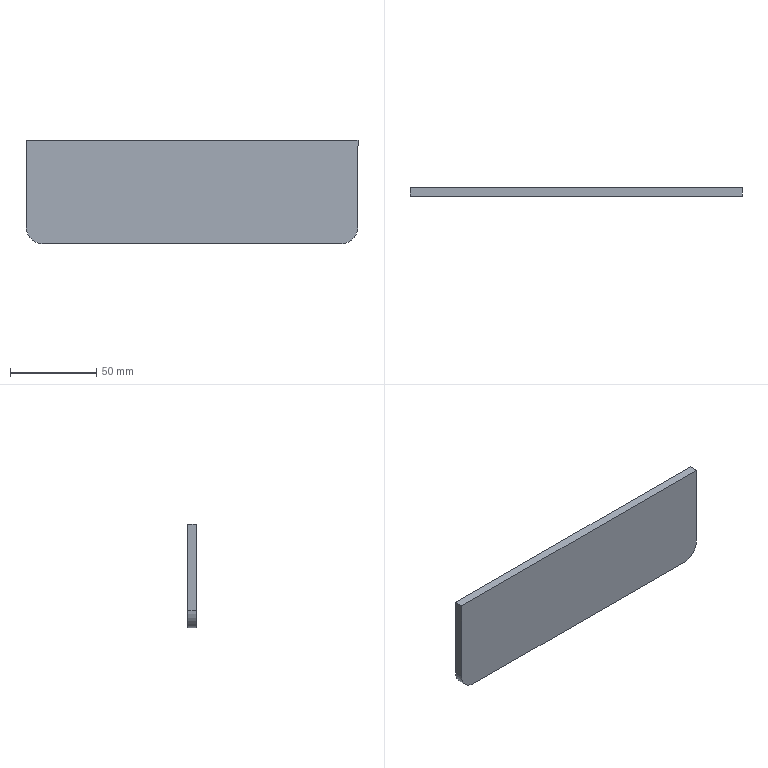Component | SolidWorks | HangingChannelAssembly-2_HangingChannelStiffener-1 | 1 solid | 8 faces | box 192 x 5 x 60 mm | volume 57385 mm3 | plane 6 | cylinder 2 | commonest cylinder face diameters 20 x2 | material Plain Carbon Steel
build123d program:
from build123d import *

# Parameters (mm, degrees)
BOSS_EXTRUDE1_DEPTH = 5


with BuildPart() as part:
    # Sketch1 → Boss-Extrude1 (new body)
    with BuildSketch(Plane.XY):
        with BuildLine():
            Line((10, 0), (182, 0))
            ThreePointArc((182, 0), (189.071, 2.929), (192, 10))
            Line((192, 10), (192, 60))
            Line((192, 60), (0, 60))
            Line((0, 60), (0, 10))
            ThreePointArc((0, 10), (2.929, 2.929), (10, 0))
        make_face()
    extrude(amount=BOSS_EXTRUDE1_DEPTH)


solid = part.part

# Placed as in the assembly
solid = solid.moved(Location((343.287, 616.049, 2029.478), (90, 0, 0)))
STEP:
#1=CARTESIAN_POINT('',(13.515,24.057,80.294));
#2=VERTEX_POINT('',#1);
#3=CARTESIAN_POINT('',(13.515,24.057,82.263));
#4=VERTEX_POINT('',#3);
#5=CARTESIAN_POINT('',(13.515,24.057,80.294));
#6=DIRECTION('',(0.,0.,1.));
#7=VECTOR('',#6,39.37);
#8=LINE('',#5,#7);
#9=EDGE_CURVE('',#2,#4,#8,.T.);
#10=ORIENTED_EDGE('',*,*,#9,.T.);
#11=CARTESIAN_POINT('',(13.515,24.254,82.263));
#12=VERTEX_POINT('',#11);
#13=CARTESIAN_POINT('',(13.515,24.254,82.263));
#14=DIRECTION('',(-0.,-1.,0.));
#15=VECTOR('',#14,39.37);
#16=LINE('',#13,#15);
#17=EDGE_CURVE('',#12,#4,#16,.T.);
#18=ORIENTED_EDGE('',*,*,#17,.F.);
#19=CARTESIAN_POINT('',(13.515,24.254,80.294));
#20=VERTEX_POINT('',#19);
#21=CARTESIAN_POINT('',(13.515,24.254,80.294));
#22=DIRECTION('',(0.,0.,1.));
#23=VECTOR('',#22,39.37);
#24=LINE('',#21,#23);
#25=EDGE_CURVE('',#20,#12,#24,.T.);
#26=ORIENTED_EDGE('',*,*,#25,.F.);
#27=CARTESIAN_POINT('',(13.515,24.254,80.294));
#28=DIRECTION('',(-0.,-1.,0.));
#29=VECTOR('',#28,39.37);
#30=LINE('',#27,#29);
#31=EDGE_CURVE('',#20,#2,#30,.T.);
#32=ORIENTED_EDGE('',*,*,#31,.T.);
#33=EDGE_LOOP('',(#10,#18,#26,#32));
#34=FACE_OUTER_BOUND('',#33,.T.);
#35=CARTESIAN_POINT('',(13.515,24.254,80.294));
#36=DIRECTION('',(1.,-0.,-0.));
#37=DIRECTION('',(0.,1.,-0.));
#38=AXIS2_PLACEMENT_3D('',#35,#36,#37);
#39=PLANE('',#38);
#40=ADVANCED_FACE('',(#34),#39,.F.);
#41=CARTESIAN_POINT('',(21.074,24.057,82.263));
#42=VERTEX_POINT('',#41);
#43=CARTESIAN_POINT('',(21.074,24.057,82.263));
#44=DIRECTION('',(1.,-0.,-0.));
#45=VECTOR('',#44,39.37);
#46=LINE('',#43,#45);
#47=EDGE_CURVE('',#4,#42,#46,.T.);
#48=ORIENTED_EDGE('',*,*,#47,.T.);
#49=CARTESIAN_POINT('',(21.074,24.254,82.263));
#50=VERTEX_POINT('',#49);
#51=CARTESIAN_POINT('',(21.074,24.254,82.263));
#52=DIRECTION('',(-0.,-1.,0.));
#53=VECTOR('',#52,39.37);
#54=LINE('',#51,#53);
#55=EDGE_CURVE('',#50,#42,#54,.T.);
#56=ORIENTED_EDGE('',*,*,#55,.F.);
#57=CARTESIAN_POINT('',(21.074,24.254,82.263));
#58=DIRECTION('',(1.,-0.,-0.));
#59=VECTOR('',#58,39.37);
#60=LINE('',#57,#59);
#61=EDGE_CURVE('',#12,#50,#60,.T.);
#62=ORIENTED_EDGE('',*,*,#61,.F.);
#63=ORIENTED_EDGE('',*,*,#17,.T.);
#64=EDGE_LOOP('',(#48,#56,#62,#63));
#65=FACE_OUTER_BOUND('',#64,.T.);
#66=CARTESIAN_POINT('',(21.074,24.254,82.263));
#67=DIRECTION('',(-0.,-0.,-1.));
#68=DIRECTION('',(-0.,-1.,0.));
#69=AXIS2_PLACEMENT_3D('',#66,#67,#68);
#70=PLANE('',#69);
#71=ADVANCED_FACE('',(#65),#70,.F.);
#72=CARTESIAN_POINT('',(21.074,24.057,80.294));
#73=VERTEX_POINT('',#72);
#74=CARTESIAN_POINT('',(21.074,24.057,80.294));
#75=DIRECTION('',(-0.,-0.,-1.));
#76=VECTOR('',#75,39.37);
#77=LINE('',#74,#76);
#78=EDGE_CURVE('',#42,#73,#77,.T.);
#79=ORIENTED_EDGE('',*,*,#78,.T.);
#80=CARTESIAN_POINT('',(21.074,24.254,80.294));
#81=VERTEX_POINT('',#80);
#82=CARTESIAN_POINT('',(21.074,24.254,80.294));
#83=DIRECTION('',(-0.,-1.,0.));
#84=VECTOR('',#83,39.37);
#85=LINE('',#82,#84);
#86=EDGE_CURVE('',#81,#73,#85,.T.);
#87=ORIENTED_EDGE('',*,*,#86,.F.);
#88=CARTESIAN_POINT('',(21.074,24.254,80.294));
#89=DIRECTION('',(-0.,-0.,-1.));
#90=VECTOR('',#89,39.37);
#91=LINE('',#88,#90);
#92=EDGE_CURVE('',#50,#81,#91,.T.);
#93=ORIENTED_EDGE('',*,*,#92,.F.);
#94=ORIENTED_EDGE('',*,*,#55,.T.);
#95=EDGE_LOOP('',(#79,#87,#93,#94));
#96=FACE_OUTER_BOUND('',#95,.T.);
#97=CARTESIAN_POINT('',(21.074,24.254,80.294));
#98=DIRECTION('',(-1.,0.,0.));
#99=DIRECTION('',(-0.,-1.,0.));
#100=AXIS2_PLACEMENT_3D('',#97,#98,#99);
#101=PLANE('',#100);
#102=ADVANCED_FACE('',(#96),#101,.F.);
#103=CARTESIAN_POINT('',(20.681,24.057,79.901));
#104=VERTEX_POINT('',#103);
#105=CARTESIAN_POINT('',(20.681,24.057,80.294));
#106=DIRECTION('',(0.,1.,-0.));
#107=DIRECTION('',(-1.,0.,0.));
#108=AXIS2_PLACEMENT_3D('',#105,#106,#107);
#109=CIRCLE('',#108,0.3937);
#110=EDGE_CURVE('',#73,#104,#109,.T.);
#111=ORIENTED_EDGE('',*,*,#110,.T.);
#112=CARTESIAN_POINT('',(20.681,24.254,79.901));
#113=VERTEX_POINT('',#112);
#114=CARTESIAN_POINT('',(20.681,24.254,79.901));
#115=DIRECTION('',(-0.,-1.,0.));
#116=VECTOR('',#115,39.37);
#117=LINE('',#114,#116);
#118=EDGE_CURVE('',#113,#104,#117,.T.);
#119=ORIENTED_EDGE('',*,*,#118,.F.);
#120=CARTESIAN_POINT('',(20.681,24.254,80.294));
#121=DIRECTION('',(0.,1.,-0.));
#122=DIRECTION('',(-1.,0.,0.));
#123=AXIS2_PLACEMENT_3D('',#120,#121,#122);
#124=CIRCLE('',#123,0.3937);
#125=EDGE_CURVE('',#81,#113,#124,.T.);
#126=ORIENTED_EDGE('',*,*,#125,.F.);
#127=ORIENTED_EDGE('',*,*,#86,.T.);
#128=EDGE_LOOP('',(#111,#119,#126,#127));
#129=FACE_OUTER_BOUND('',#128,.T.);
#130=CARTESIAN_POINT('',(20.681,24.254,80.294));
#131=DIRECTION('',(-0.,-1.,0.));
#132=DIRECTION('',(1.,0.,0.));
#133=AXIS2_PLACEMENT_3D('',#130,#131,#132);
#134=CYLINDRICAL_SURFACE('',#133,0.3937);
#135=ADVANCED_FACE('',(#129),#134,.T.);
#136=CARTESIAN_POINT('',(13.909,24.057,79.901));
#137=VERTEX_POINT('',#136);
#138=CARTESIAN_POINT('',(20.681,24.057,79.901));
#139=DIRECTION('',(-1.,0.,0.));
#140=VECTOR('',#139,39.37);
#141=LINE('',#138,#140);
#142=EDGE_CURVE('',#104,#137,#141,.T.);
#143=ORIENTED_EDGE('',*,*,#142,.T.);
#144=CARTESIAN_POINT('',(13.909,24.254,79.901));
#145=VERTEX_POINT('',#144);
#146=CARTESIAN_POINT('',(13.909,24.254,79.901));
#147=DIRECTION('',(-0.,-1.,0.));
#148=VECTOR('',#147,39.37);
#149=LINE('',#146,#148);
#150=EDGE_CURVE('',#145,#137,#149,.T.);
#151=ORIENTED_EDGE('',*,*,#150,.F.);
#152=CARTESIAN_POINT('',(20.681,24.254,79.901));
#153=DIRECTION('',(-1.,0.,0.));
#154=VECTOR('',#153,39.37);
#155=LINE('',#152,#154);
#156=EDGE_CURVE('',#113,#145,#155,.T.);
#157=ORIENTED_EDGE('',*,*,#156,.F.);
#158=ORIENTED_EDGE('',*,*,#118,.T.);
#159=EDGE_LOOP('',(#143,#151,#157,#158));
#160=FACE_OUTER_BOUND('',#159,.T.);
#161=CARTESIAN_POINT('',(20.681,24.254,79.901));
#162=DIRECTION('',(0.,0.,1.));
#163=DIRECTION('',(0.,1.,-0.));
#164=AXIS2_PLACEMENT_3D('',#161,#162,#163);
#165=PLANE('',#164);
#166=ADVANCED_FACE('',(#160),#165,.F.);
#167=CARTESIAN_POINT('',(13.909,24.057,80.294));
#168=DIRECTION('',(0.,1.,-0.));
#169=DIRECTION('',(1.,0.,0.));
#170=AXIS2_PLACEMENT_3D('',#167,#168,#169);
#171=CIRCLE('',#170,0.3937);
#172=EDGE_CURVE('',#137,#2,#171,.T.);
#173=ORIENTED_EDGE('',*,*,#172,.T.);
#174=ORIENTED_EDGE('',*,*,#31,.F.);
#175=CARTESIAN_POINT('',(13.909,24.254,80.294));
#176=DIRECTION('',(0.,1.,-0.));
#177=DIRECTION('',(1.,0.,0.));
#178=AXIS2_PLACEMENT_3D('',#175,#176,#177);
#179=CIRCLE('',#178,0.3937);
#180=EDGE_CURVE('',#145,#20,#179,.T.);
#181=ORIENTED_EDGE('',*,*,#180,.F.);
#182=ORIENTED_EDGE('',*,*,#150,.T.);
#183=EDGE_LOOP('',(#173,#174,#181,#182));
#184=FACE_OUTER_BOUND('',#183,.T.);
#185=CARTESIAN_POINT('',(13.909,24.254,80.294));
#186=DIRECTION('',(-0.,-1.,0.));
#187=DIRECTION('',(1.,0.,0.));
#188=AXIS2_PLACEMENT_3D('',#185,#186,#187);
#189=CYLINDRICAL_SURFACE('',#188,0.3937);
#190=ADVANCED_FACE('',(#184),#189,.T.);
#191=ORIENTED_EDGE('',*,*,#25,.T.);
#192=ORIENTED_EDGE('',*,*,#61,.T.);
#193=ORIENTED_EDGE('',*,*,#92,.T.);
#194=ORIENTED_EDGE('',*,*,#125,.T.);
#195=ORIENTED_EDGE('',*,*,#156,.T.);
#196=ORIENTED_EDGE('',*,*,#180,.T.);
#197=EDGE_LOOP('',(#191,#192,#193,#194,#195,#196));
#198=FACE_OUTER_BOUND('',#197,.T.);
#199=CARTESIAN_POINT('',(20.681,24.254,80.294));
#200=DIRECTION('',(0.,1.,-0.));
#201=DIRECTION('',(-1.,0.,0.));
#202=AXIS2_PLACEMENT_3D('',#199,#200,#201);
#203=PLANE('',#202);
#204=ADVANCED_FACE('',(#198),#203,.T.);
#205=ORIENTED_EDGE('',*,*,#9,.F.);
#206=ORIENTED_EDGE('',*,*,#172,.F.);
#207=ORIENTED_EDGE('',*,*,#142,.F.);
#208=ORIENTED_EDGE('',*,*,#110,.F.);
#209=ORIENTED_EDGE('',*,*,#78,.F.);
#210=ORIENTED_EDGE('',*,*,#47,.F.);
#211=EDGE_LOOP('',(#205,#206,#207,#208,#209,#210));
#212=FACE_OUTER_BOUND('',#211,.T.);
#213=CARTESIAN_POINT('',(20.681,24.057,80.294));
#214=DIRECTION('',(0.,1.,-0.));
#215=DIRECTION('',(-1.,0.,0.));
#216=AXIS2_PLACEMENT_3D('',#213,#214,#215);
#217=PLANE('',#216);
#218=ADVANCED_FACE('',(#212),#217,.F.);
#219=CLOSED_SHELL('',(#40,#71,#102,#135,#166,#190,#204,#218));
#220=MANIFOLD_SOLID_BREP('',#219);
#221=CARTESIAN_POINT('',(0.,0.,0.));
#222=DIRECTION('',(0.,0.,1.));
#223=DIRECTION('',(1.,0.,0.));
#224=AXIS2_PLACEMENT_3D('',#221,#222,#223);
#225=(LENGTH_UNIT()NAMED_UNIT(*)SI_UNIT($,.METRE.));
#226=LENGTH_MEASURE_WITH_UNIT(LENGTH_MEASURE(0.0254),#225);
#227=DIMENSIONAL_EXPONENTS(1.,0.,0.,0.,0.,0.,0.);
#228=(CONVERSION_BASED_UNIT('',#226)LENGTH_UNIT()NAMED_UNIT(#227));
#229=UNCERTAINTY_MEASURE_WITH_UNIT(LENGTH_MEASURE(0.00001),#228,'','');
#230=(NAMED_UNIT(*)PLANE_ANGLE_UNIT()SI_UNIT($,.RADIAN.));
#231=(NAMED_UNIT(*)SI_UNIT($,.STERADIAN.)SOLID_ANGLE_UNIT());
#232=(GEOMETRIC_REPRESENTATION_CONTEXT(3)GLOBAL_UNCERTAINTY_ASSIGNED_CONTEXT((#229))GLOBAL_UNIT_ASSIGNED_CONTEXT((#228,#230,#231))REPRESENTATION_CONTEXT('',''));
#233=ADVANCED_BREP_SHAPE_REPRESENTATION('',(#220,#224),#232);
#234=COLOUR_RGB('',0.7922,0.8196,0.9333);
#235=FILL_AREA_STYLE_COLOUR('',#234);
#236=FILL_AREA_STYLE('',(#235));
#237=SURFACE_STYLE_FILL_AREA(#236);
#238=SURFACE_SIDE_STYLE('',(#237));
#239=SURFACE_STYLE_USAGE(.BOTH.,#238);
#240=PRESENTATION_STYLE_ASSIGNMENT((#239));
#241=STYLED_ITEM('',(#240),#220);
#242=(LENGTH_UNIT()NAMED_UNIT(*)SI_UNIT($,.METRE.));
#243=LENGTH_MEASURE_WITH_UNIT(LENGTH_MEASURE(0.0254),#242);
#244=DIMENSIONAL_EXPONENTS(1.,0.,0.,0.,0.,0.,0.);
#245=(CONVERSION_BASED_UNIT('',#243)LENGTH_UNIT()NAMED_UNIT(#244));
#246=UNCERTAINTY_MEASURE_WITH_UNIT(LENGTH_MEASURE(0.00001),#245,'','');
#247=(NAMED_UNIT(*)PLANE_ANGLE_UNIT()SI_UNIT($,.RADIAN.));
#248=(NAMED_UNIT(*)SI_UNIT($,.STERADIAN.)SOLID_ANGLE_UNIT());
#249=(GEOMETRIC_REPRESENTATION_CONTEXT(3)GLOBAL_UNCERTAINTY_ASSIGNED_CONTEXT((#246))GLOBAL_UNIT_ASSIGNED_CONTEXT((#245,#247,#248))REPRESENTATION_CONTEXT('',''));
#250=MECHANICAL_DESIGN_GEOMETRIC_PRESENTATION_REPRESENTATION('',(#241),#249);
#251=PRESENTATION_LAYER_ASSIGNMENT('','',(#241));